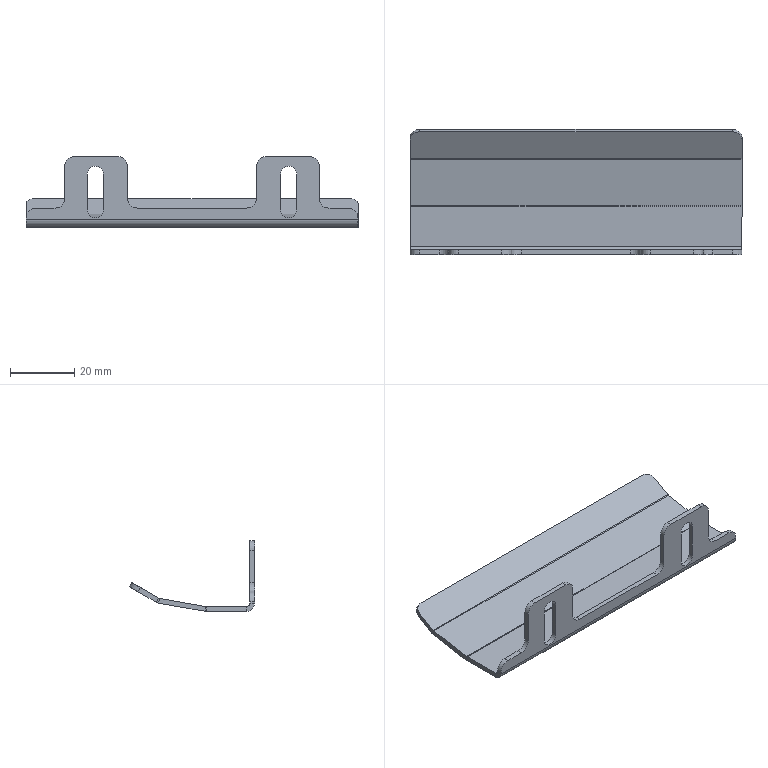Component | SolidWorks | XM-02-006A1-1 | 1 solid | 58 faces | volume 7459 mm3 | plane 36 | cylinder 22 | commonest cylinder face diameters 6 x12 5 x7 2 x3 | material SUS304